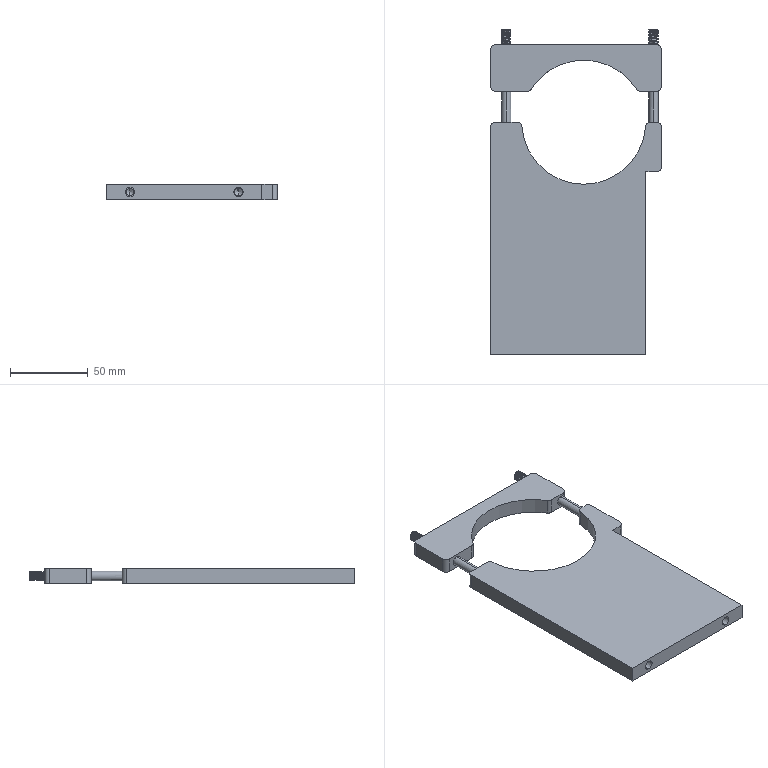Component | SolidWorks | PipeLockPlate.1-1 | 4 solids | 139 faces | volume 151389 mm3 | cylinder 107 | plane 24 | cone 4 | spline 4 | commonest cylinder face diameters 6 x97 5 x4 6.5 x4 80 x2